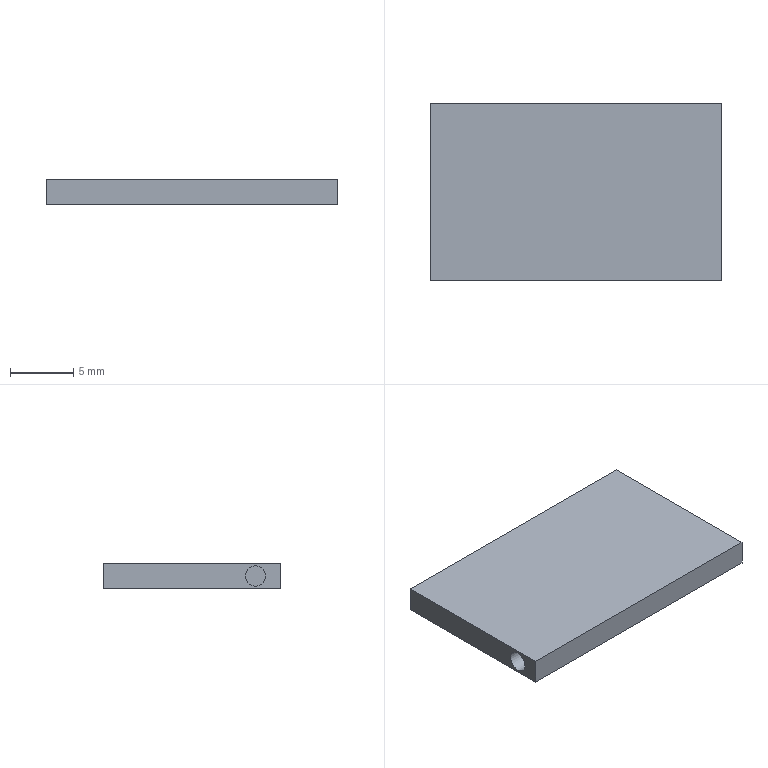Component | NX | CONNECTING_RECT_2 | 1 solid | 10 faces | box 23 x 14 x 2 mm | volume 636 mm3 | plane 8 | cylinder 2 | commonest cylinder face diameters 1.6 x2
STEP:
#1=CARTESIAN_POINT('',(0.,0.,0.));
#2=DIRECTION('',(0.,0.,1.));
#3=DIRECTION('',(1.,0.,0.));
#4=AXIS2_PLACEMENT_3D('',#1,#2,#3);
#5=CARTESIAN_POINT('',(-11.5,-4.375,30.));
#6=VERTEX_POINT('',#5);
#7=CARTESIAN_POINT('',(-11.5,-3.575,30.));
#8=DIRECTION('',(1.,0.,0.));
#9=DIRECTION('',(0.,-1.,0.));
#10=AXIS2_PLACEMENT_3D('',#7,#8,#9);
#11=CIRCLE('',#10,0.8);
#12=CARTESIAN_POINT('',(-11.5,8.425,29.));
#13=DIRECTION('',(-1.,0.,0.));
#14=DIRECTION('',(0.,0.,1.));
#15=AXIS2_PLACEMENT_3D('',#12,#13,#14);
#16=PLANE('',#15);
#17=CARTESIAN_POINT('',(1.,-12.8));
#18=CARTESIAN_POINT('',(-0.3856,-12.8));
#19=CARTESIAN_POINT('',(0.3072,-11.6));
#20=CARTESIAN_POINT('',(1.,-10.4));
#21=CARTESIAN_POINT('',(1.693,-11.6));
#22=CARTESIAN_POINT('',(2.386,-12.8));
#23=CARTESIAN_POINT('',(1.,-12.8));
#24=(BOUNDED_CURVE()B_SPLINE_CURVE(2,(#17,#18,#19,#20,#21,#22,#23),.UNSPECIFIED.,.T.,.F.)B_SPLINE_CURVE_WITH_KNOTS((1,2,2,2,2,1),(-2.094,0.,2.094,4.189,6.283,8.378),.UNSPECIFIED.)CURVE()GEOMETRIC_REPRESENTATION_ITEM()RATIONAL_B_SPLINE_CURVE((1.,0.5,1.,0.5,1.,0.5,1.))REPRESENTATION_ITEM(''));
#25=(GEOMETRIC_REPRESENTATION_CONTEXT(2)PARAMETRIC_REPRESENTATION_CONTEXT()REPRESENTATION_CONTEXT('',''));
#26=DEFINITIONAL_REPRESENTATION('',(#24),#25);
#27=PCURVE('',#16,#26);
#28=CARTESIAN_POINT('',(-9.5,-3.575,30.));
#29=DIRECTION('',(-1.,0.,0.));
#30=DIRECTION('',(0.,0.,1.));
#31=AXIS2_PLACEMENT_3D('',#28,#29,#30);
#32=CYLINDRICAL_SURFACE('',#31,0.8);
#33=CARTESIAN_POINT('',(10.996,2.));
#34=DIRECTION('',(-1.,0.));
#35=VECTOR('',#34,1.);
#36=LINE('',#33,#35);
#37=(GEOMETRIC_REPRESENTATION_CONTEXT(2)PARAMETRIC_REPRESENTATION_CONTEXT()REPRESENTATION_CONTEXT('',''));
#38=DEFINITIONAL_REPRESENTATION('',(#36),#37);
#39=PCURVE('',#32,#38);
#40=SURFACE_CURVE('',#11,(#27,#39),.PCURVE_S1.);
#41=EDGE_CURVE('',#6,#6,#40,.T.);
#42=ORIENTED_EDGE('',*,*,#41,.T.);
#43=EDGE_LOOP('',(#42));
#44=FACE_BOUND('',#43,.T.);
#45=CARTESIAN_POINT('',(-11.5,8.425,31.));
#46=VERTEX_POINT('',#45);
#47=CARTESIAN_POINT('',(-11.5,-5.575,31.));
#48=VERTEX_POINT('',#47);
#49=CARTESIAN_POINT('',(-11.5,8.425,31.));
#50=DIRECTION('',(0.,-1.,0.));
#51=VECTOR('',#50,1.);
#52=LINE('',#49,#51);
#53=CARTESIAN_POINT('',(2.,0.));
#54=DIRECTION('',(0.,-1.));
#55=VECTOR('',#54,1.);
#56=LINE('',#53,#55);
#57=(GEOMETRIC_REPRESENTATION_CONTEXT(2)PARAMETRIC_REPRESENTATION_CONTEXT()REPRESENTATION_CONTEXT('',''));
#58=DEFINITIONAL_REPRESENTATION('',(#56),#57);
#59=PCURVE('',#16,#58);
#60=CARTESIAN_POINT('',(6.5,1.925,31.));
#61=DIRECTION('',(0.,0.,1.));
#62=DIRECTION('',(1.,0.,0.));
#63=AXIS2_PLACEMENT_3D('',#60,#61,#62);
#64=PLANE('',#63);
#65=CARTESIAN_POINT('',(-18.,6.5));
#66=DIRECTION('',(0.,-1.));
#67=VECTOR('',#66,1.);
#68=LINE('',#65,#67);
#69=(GEOMETRIC_REPRESENTATION_CONTEXT(2)PARAMETRIC_REPRESENTATION_CONTEXT()REPRESENTATION_CONTEXT('',''));
#70=DEFINITIONAL_REPRESENTATION('',(#68),#69);
#71=PCURVE('',#64,#70);
#72=SURFACE_CURVE('',#52,(#59,#71),.PCURVE_S1.);
#73=EDGE_CURVE('',#46,#48,#72,.T.);
#74=ORIENTED_EDGE('',*,*,#73,.F.);
#75=CARTESIAN_POINT('',(-11.5,8.425,29.));
#76=VERTEX_POINT('',#75);
#77=CARTESIAN_POINT('',(-11.5,8.425,29.));
#78=DIRECTION('',(0.,0.,1.));
#79=VECTOR('',#78,1.);
#80=LINE('',#77,#79);
#81=CARTESIAN_POINT('',(0.,0.));
#82=DIRECTION('',(1.,0.));
#83=VECTOR('',#82,1.);
#84=LINE('',#81,#83);
#85=(GEOMETRIC_REPRESENTATION_CONTEXT(2)PARAMETRIC_REPRESENTATION_CONTEXT()REPRESENTATION_CONTEXT('',''));
#86=DEFINITIONAL_REPRESENTATION('',(#84),#85);
#87=PCURVE('',#16,#86);
#88=CARTESIAN_POINT('',(11.5,8.425,29.));
#89=DIRECTION('',(-0.,1.,0.));
#90=DIRECTION('',(-1.,-0.,0.));
#91=AXIS2_PLACEMENT_3D('',#88,#89,#90);
#92=PLANE('',#91);
#93=CARTESIAN_POINT('',(23.,0.));
#94=DIRECTION('',(0.,1.));
#95=VECTOR('',#94,1.);
#96=LINE('',#93,#95);
#97=(GEOMETRIC_REPRESENTATION_CONTEXT(2)PARAMETRIC_REPRESENTATION_CONTEXT()REPRESENTATION_CONTEXT('',''));
#98=DEFINITIONAL_REPRESENTATION('',(#96),#97);
#99=PCURVE('',#92,#98);
#100=SURFACE_CURVE('',#80,(#87,#99),.PCURVE_S1.);
#101=EDGE_CURVE('',#76,#46,#100,.T.);
#102=ORIENTED_EDGE('',*,*,#101,.F.);
#103=CARTESIAN_POINT('',(-11.5,-5.575,29.));
#104=VERTEX_POINT('',#103);
#105=CARTESIAN_POINT('',(-11.5,8.425,29.));
#106=DIRECTION('',(0.,-1.,0.));
#107=VECTOR('',#106,1.);
#108=LINE('',#105,#107);
#109=CARTESIAN_POINT('',(0.,0.));
#110=DIRECTION('',(0.,-1.));
#111=VECTOR('',#110,1.);
#112=LINE('',#109,#111);
#113=(GEOMETRIC_REPRESENTATION_CONTEXT(2)PARAMETRIC_REPRESENTATION_CONTEXT()REPRESENTATION_CONTEXT('',''));
#114=DEFINITIONAL_REPRESENTATION('',(#112),#113);
#115=PCURVE('',#16,#114);
#116=CARTESIAN_POINT('',(6.5,1.925,29.));
#117=DIRECTION('',(0.,0.,1.));
#118=DIRECTION('',(1.,0.,0.));
#119=AXIS2_PLACEMENT_3D('',#116,#117,#118);
#120=PLANE('',#119);
#121=CARTESIAN_POINT('',(-18.,6.5));
#122=DIRECTION('',(0.,-1.));
#123=VECTOR('',#122,1.);
#124=LINE('',#121,#123);
#125=(GEOMETRIC_REPRESENTATION_CONTEXT(2)PARAMETRIC_REPRESENTATION_CONTEXT()REPRESENTATION_CONTEXT('',''));
#126=DEFINITIONAL_REPRESENTATION('',(#124),#125);
#127=PCURVE('',#120,#126);
#128=SURFACE_CURVE('',#108,(#115,#127),.PCURVE_S1.);
#129=EDGE_CURVE('',#76,#104,#128,.T.);
#130=ORIENTED_EDGE('',*,*,#129,.T.);
#131=CARTESIAN_POINT('',(-11.5,-5.575,29.));
#132=DIRECTION('',(0.,0.,1.));
#133=VECTOR('',#132,1.);
#134=LINE('',#131,#133);
#135=CARTESIAN_POINT('',(0.,-14.));
#136=DIRECTION('',(1.,0.));
#137=VECTOR('',#136,1.);
#138=LINE('',#135,#137);
#139=(GEOMETRIC_REPRESENTATION_CONTEXT(2)PARAMETRIC_REPRESENTATION_CONTEXT()REPRESENTATION_CONTEXT('',''));
#140=DEFINITIONAL_REPRESENTATION('',(#138),#139);
#141=PCURVE('',#16,#140);
#142=CARTESIAN_POINT('',(-11.5,-5.575,29.));
#143=DIRECTION('',(0.,-1.,0.));
#144=DIRECTION('',(1.,0.,0.));
#145=AXIS2_PLACEMENT_3D('',#142,#143,#144);
#146=PLANE('',#145);
#147=CARTESIAN_POINT('',(0.,0.));
#148=DIRECTION('',(0.,1.));
#149=VECTOR('',#148,1.);
#150=LINE('',#147,#149);
#151=(GEOMETRIC_REPRESENTATION_CONTEXT(2)PARAMETRIC_REPRESENTATION_CONTEXT()REPRESENTATION_CONTEXT('',''));
#152=DEFINITIONAL_REPRESENTATION('',(#150),#151);
#153=PCURVE('',#146,#152);
#154=SURFACE_CURVE('',#134,(#141,#153),.PCURVE_S1.);
#155=EDGE_CURVE('',#104,#48,#154,.T.);
#156=ORIENTED_EDGE('',*,*,#155,.T.);
#157=EDGE_LOOP('',(#74,#102,#130,#156));
#158=FACE_BOUND('',#157,.T.);
#159=ADVANCED_FACE('',(#44,#158),#16,.T.);
#160=CARTESIAN_POINT('',(11.5,-5.575,31.));
#161=VERTEX_POINT('',#160);
#162=CARTESIAN_POINT('',(-11.5,-5.575,31.));
#163=DIRECTION('',(1.,0.,0.));
#164=VECTOR('',#163,1.);
#165=LINE('',#162,#164);
#166=CARTESIAN_POINT('',(0.,2.));
#167=DIRECTION('',(1.,0.));
#168=VECTOR('',#167,1.);
#169=LINE('',#166,#168);
#170=(GEOMETRIC_REPRESENTATION_CONTEXT(2)PARAMETRIC_REPRESENTATION_CONTEXT()REPRESENTATION_CONTEXT('',''));
#171=DEFINITIONAL_REPRESENTATION('',(#169),#170);
#172=PCURVE('',#146,#171);
#173=CARTESIAN_POINT('',(-18.,-7.5));
#174=DIRECTION('',(1.,0.));
#175=VECTOR('',#174,1.);
#176=LINE('',#173,#175);
#177=(GEOMETRIC_REPRESENTATION_CONTEXT(2)PARAMETRIC_REPRESENTATION_CONTEXT()REPRESENTATION_CONTEXT('',''));
#178=DEFINITIONAL_REPRESENTATION('',(#176),#177);
#179=PCURVE('',#64,#178);
#180=SURFACE_CURVE('',#165,(#172,#179),.PCURVE_S1.);
#181=EDGE_CURVE('',#48,#161,#180,.T.);
#182=ORIENTED_EDGE('',*,*,#181,.F.);
#183=ORIENTED_EDGE('',*,*,#155,.F.);
#184=CARTESIAN_POINT('',(11.5,-5.575,29.));
#185=VERTEX_POINT('',#184);
#186=CARTESIAN_POINT('',(-11.5,-5.575,29.));
#187=DIRECTION('',(1.,0.,0.));
#188=VECTOR('',#187,1.);
#189=LINE('',#186,#188);
#190=CARTESIAN_POINT('',(0.,0.));
#191=DIRECTION('',(1.,0.));
#192=VECTOR('',#191,1.);
#193=LINE('',#190,#192);
#194=(GEOMETRIC_REPRESENTATION_CONTEXT(2)PARAMETRIC_REPRESENTATION_CONTEXT()REPRESENTATION_CONTEXT('',''));
#195=DEFINITIONAL_REPRESENTATION('',(#193),#194);
#196=PCURVE('',#146,#195);
#197=CARTESIAN_POINT('',(-18.,-7.5));
#198=DIRECTION('',(1.,0.));
#199=VECTOR('',#198,1.);
#200=LINE('',#197,#199);
#201=(GEOMETRIC_REPRESENTATION_CONTEXT(2)PARAMETRIC_REPRESENTATION_CONTEXT()REPRESENTATION_CONTEXT('',''));
#202=DEFINITIONAL_REPRESENTATION('',(#200),#201);
#203=PCURVE('',#120,#202);
#204=SURFACE_CURVE('',#189,(#196,#203),.PCURVE_S1.);
#205=EDGE_CURVE('',#104,#185,#204,.T.);
#206=ORIENTED_EDGE('',*,*,#205,.T.);
#207=CARTESIAN_POINT('',(11.5,-5.575,29.));
#208=DIRECTION('',(0.,0.,1.));
#209=VECTOR('',#208,1.);
#210=LINE('',#207,#209);
#211=CARTESIAN_POINT('',(23.,0.));
#212=DIRECTION('',(0.,1.));
#213=VECTOR('',#212,1.);
#214=LINE('',#211,#213);
#215=(GEOMETRIC_REPRESENTATION_CONTEXT(2)PARAMETRIC_REPRESENTATION_CONTEXT()REPRESENTATION_CONTEXT('',''));
#216=DEFINITIONAL_REPRESENTATION('',(#214),#215);
#217=PCURVE('',#146,#216);
#218=CARTESIAN_POINT('',(11.5,-5.575,29.));
#219=DIRECTION('',(1.,0.,0.));
#220=DIRECTION('',(-0.,1.,0.));
#221=AXIS2_PLACEMENT_3D('',#218,#219,#220);
#222=PLANE('',#221);
#223=CARTESIAN_POINT('',(0.,0.));
#224=DIRECTION('',(0.,1.));
#225=VECTOR('',#224,1.);
#226=LINE('',#223,#225);
#227=(GEOMETRIC_REPRESENTATION_CONTEXT(2)PARAMETRIC_REPRESENTATION_CONTEXT()REPRESENTATION_CONTEXT('',''));
#228=DEFINITIONAL_REPRESENTATION('',(#226),#227);
#229=PCURVE('',#222,#228);
#230=SURFACE_CURVE('',#210,(#217,#229),.PCURVE_S1.);
#231=EDGE_CURVE('',#185,#161,#230,.T.);
#232=ORIENTED_EDGE('',*,*,#231,.T.);
#233=EDGE_LOOP('',(#182,#183,#206,#232));
#234=FACE_BOUND('',#233,.T.);
#235=ADVANCED_FACE('',(#234),#146,.T.);
#236=CARTESIAN_POINT('',(11.5,7.225,30.));
#237=VERTEX_POINT('',#236);
#238=CARTESIAN_POINT('',(11.5,6.425,30.));
#239=DIRECTION('',(1.,0.,0.));
#240=DIRECTION('',(0.,1.,0.));
#241=AXIS2_PLACEMENT_3D('',#238,#239,#240);
#242=CIRCLE('',#241,0.8);
#243=CARTESIAN_POINT('',(12.,1.));
#244=DIRECTION('',(1.,0.));
#245=AXIS2_PLACEMENT_2D('',#243,#244);
#246=CIRCLE('',#245,0.8);
#247=(GEOMETRIC_REPRESENTATION_CONTEXT(2)PARAMETRIC_REPRESENTATION_CONTEXT()REPRESENTATION_CONTEXT('',''));
#248=DEFINITIONAL_REPRESENTATION('',(#246),#247);
#249=PCURVE('',#222,#248);
#250=CARTESIAN_POINT('',(9.5,6.425,30.));
#251=DIRECTION('',(1.,0.,0.));
#252=DIRECTION('',(0.,0.,-1.));
#253=AXIS2_PLACEMENT_3D('',#250,#251,#252);
#254=CYLINDRICAL_SURFACE('',#253,0.8);
#255=CARTESIAN_POINT('',(1.571,2.));
#256=DIRECTION('',(1.,0.));
#257=VECTOR('',#256,1.);
#258=LINE('',#255,#257);
#259=(GEOMETRIC_REPRESENTATION_CONTEXT(2)PARAMETRIC_REPRESENTATION_CONTEXT()REPRESENTATION_CONTEXT('',''));
#260=DEFINITIONAL_REPRESENTATION('',(#258),#259);
#261=PCURVE('',#254,#260);
#262=SURFACE_CURVE('',#242,(#249,#261),.PCURVE_S1.);
#263=EDGE_CURVE('',#237,#237,#262,.T.);
#264=ORIENTED_EDGE('',*,*,#263,.F.);
#265=EDGE_LOOP('',(#264));
#266=FACE_BOUND('',#265,.T.);
#267=CARTESIAN_POINT('',(11.5,8.425,31.));
#268=VERTEX_POINT('',#267);
#269=CARTESIAN_POINT('',(11.5,-5.575,31.));
#270=DIRECTION('',(-0.,1.,0.));
#271=VECTOR('',#270,1.);
#272=LINE('',#269,#271);
#273=CARTESIAN_POINT('',(0.,2.));
#274=DIRECTION('',(1.,0.));
#275=VECTOR('',#274,1.);
#276=LINE('',#273,#275);
#277=(GEOMETRIC_REPRESENTATION_CONTEXT(2)PARAMETRIC_REPRESENTATION_CONTEXT()REPRESENTATION_CONTEXT('',''));
#278=DEFINITIONAL_REPRESENTATION('',(#276),#277);
#279=PCURVE('',#222,#278);
#280=CARTESIAN_POINT('',(5.,-7.5));
#281=DIRECTION('',(-0.,1.));
#282=VECTOR('',#281,1.);
#283=LINE('',#280,#282);
#284=(GEOMETRIC_REPRESENTATION_CONTEXT(2)PARAMETRIC_REPRESENTATION_CONTEXT()REPRESENTATION_CONTEXT('',''));
#285=DEFINITIONAL_REPRESENTATION('',(#283),#284);
#286=PCURVE('',#64,#285);
#287=SURFACE_CURVE('',#272,(#279,#286),.PCURVE_S1.);
#288=EDGE_CURVE('',#161,#268,#287,.T.);
#289=ORIENTED_EDGE('',*,*,#288,.F.);
#290=ORIENTED_EDGE('',*,*,#231,.F.);
#291=CARTESIAN_POINT('',(11.5,8.425,29.));
#292=VERTEX_POINT('',#291);
#293=CARTESIAN_POINT('',(11.5,-5.575,29.));
#294=DIRECTION('',(-0.,1.,0.));
#295=VECTOR('',#294,1.);
#296=LINE('',#293,#295);
#297=CARTESIAN_POINT('',(0.,0.));
#298=DIRECTION('',(1.,0.));
#299=VECTOR('',#298,1.);
#300=LINE('',#297,#299);
#301=(GEOMETRIC_REPRESENTATION_CONTEXT(2)PARAMETRIC_REPRESENTATION_CONTEXT()REPRESENTATION_CONTEXT('',''));
#302=DEFINITIONAL_REPRESENTATION('',(#300),#301);
#303=PCURVE('',#222,#302);
#304=CARTESIAN_POINT('',(5.,-7.5));
#305=DIRECTION('',(-0.,1.));
#306=VECTOR('',#305,1.);
#307=LINE('',#304,#306);
#308=(GEOMETRIC_REPRESENTATION_CONTEXT(2)PARAMETRIC_REPRESENTATION_CONTEXT()REPRESENTATION_CONTEXT('',''));
#309=DEFINITIONAL_REPRESENTATION('',(#307),#308);
#310=PCURVE('',#120,#309);
#311=SURFACE_CURVE('',#296,(#303,#310),.PCURVE_S1.);
#312=EDGE_CURVE('',#185,#292,#311,.T.);
#313=ORIENTED_EDGE('',*,*,#312,.T.);
#314=CARTESIAN_POINT('',(11.5,8.425,29.));
#315=DIRECTION('',(0.,0.,1.));
#316=VECTOR('',#315,1.);
#317=LINE('',#314,#316);
#318=CARTESIAN_POINT('',(14.,0.));
#319=DIRECTION('',(0.,1.));
#320=VECTOR('',#319,1.);
#321=LINE('',#318,#320);
#322=(GEOMETRIC_REPRESENTATION_CONTEXT(2)PARAMETRIC_REPRESENTATION_CONTEXT()REPRESENTATION_CONTEXT('',''));
#323=DEFINITIONAL_REPRESENTATION('',(#321),#322);
#324=PCURVE('',#222,#323);
#325=CARTESIAN_POINT('',(0.,0.));
#326=DIRECTION('',(0.,1.));
#327=VECTOR('',#326,1.);
#328=LINE('',#325,#327);
#329=(GEOMETRIC_REPRESENTATION_CONTEXT(2)PARAMETRIC_REPRESENTATION_CONTEXT()REPRESENTATION_CONTEXT('',''));
#330=DEFINITIONAL_REPRESENTATION('',(#328),#329);
#331=PCURVE('',#92,#330);
#332=SURFACE_CURVE('',#317,(#324,#331),.PCURVE_S1.);
#333=EDGE_CURVE('',#292,#268,#332,.T.);
#334=ORIENTED_EDGE('',*,*,#333,.T.);
#335=EDGE_LOOP('',(#289,#290,#313,#334));
#336=FACE_BOUND('',#335,.T.);
#337=ADVANCED_FACE('',(#266,#336),#222,.T.);
#338=CARTESIAN_POINT('',(11.5,8.425,31.));
#339=DIRECTION('',(-1.,-0.,0.));
#340=VECTOR('',#339,1.);
#341=LINE('',#338,#340);
#342=CARTESIAN_POINT('',(0.,2.));
#343=DIRECTION('',(1.,0.));
#344=VECTOR('',#343,1.);
#345=LINE('',#342,#344);
#346=(GEOMETRIC_REPRESENTATION_CONTEXT(2)PARAMETRIC_REPRESENTATION_CONTEXT()REPRESENTATION_CONTEXT('',''));
#347=DEFINITIONAL_REPRESENTATION('',(#345),#346);
#348=PCURVE('',#92,#347);
#349=CARTESIAN_POINT('',(5.,6.5));
#350=DIRECTION('',(-1.,-0.));
#351=VECTOR('',#350,1.);
#352=LINE('',#349,#351);
#353=(GEOMETRIC_REPRESENTATION_CONTEXT(2)PARAMETRIC_REPRESENTATION_CONTEXT()REPRESENTATION_CONTEXT('',''));
#354=DEFINITIONAL_REPRESENTATION('',(#352),#353);
#355=PCURVE('',#64,#354);
#356=SURFACE_CURVE('',#341,(#348,#355),.PCURVE_S1.);
#357=EDGE_CURVE('',#268,#46,#356,.T.);
#358=ORIENTED_EDGE('',*,*,#357,.F.);
#359=ORIENTED_EDGE('',*,*,#333,.F.);
#360=CARTESIAN_POINT('',(11.5,8.425,29.));
#361=DIRECTION('',(-1.,-0.,0.));
#362=VECTOR('',#361,1.);
#363=LINE('',#360,#362);
#364=CARTESIAN_POINT('',(0.,0.));
#365=DIRECTION('',(1.,0.));
#366=VECTOR('',#365,1.);
#367=LINE('',#364,#366);
#368=(GEOMETRIC_REPRESENTATION_CONTEXT(2)PARAMETRIC_REPRESENTATION_CONTEXT()REPRESENTATION_CONTEXT('',''));
#369=DEFINITIONAL_REPRESENTATION('',(#367),#368);
#370=PCURVE('',#92,#369);
#371=CARTESIAN_POINT('',(5.,6.5));
#372=DIRECTION('',(-1.,-0.));
#373=VECTOR('',#372,1.);
#374=LINE('',#371,#373);
#375=(GEOMETRIC_REPRESENTATION_CONTEXT(2)PARAMETRIC_REPRESENTATION_CONTEXT()REPRESENTATION_CONTEXT('',''));
#376=DEFINITIONAL_REPRESENTATION('',(#374),#375);
#377=PCURVE('',#120,#376);
#378=SURFACE_CURVE('',#363,(#370,#377),.PCURVE_S1.);
#379=EDGE_CURVE('',#292,#76,#378,.T.);
#380=ORIENTED_EDGE('',*,*,#379,.T.);
#381=ORIENTED_EDGE('',*,*,#101,.T.);
#382=EDGE_LOOP('',(#358,#359,#380,#381));
#383=FACE_BOUND('',#382,.T.);
#384=ADVANCED_FACE('',(#383),#92,.T.);
#385=ORIENTED_EDGE('',*,*,#129,.F.);
#386=ORIENTED_EDGE('',*,*,#379,.F.);
#387=ORIENTED_EDGE('',*,*,#312,.F.);
#388=ORIENTED_EDGE('',*,*,#205,.F.);
#389=EDGE_LOOP('',(#385,#386,#387,#388));
#390=FACE_BOUND('',#389,.T.);
#391=ADVANCED_FACE('',(#390),#120,.F.);
#392=ORIENTED_EDGE('',*,*,#73,.T.);
#393=ORIENTED_EDGE('',*,*,#181,.T.);
#394=ORIENTED_EDGE('',*,*,#288,.T.);
#395=ORIENTED_EDGE('',*,*,#357,.T.);
#396=EDGE_LOOP('',(#392,#393,#394,#395));
#397=FACE_BOUND('',#396,.T.);
#398=ADVANCED_FACE('',(#397),#64,.T.);
#399=CARTESIAN_POINT('',(9.5,7.225,30.));
#400=VERTEX_POINT('',#399);
#401=CARTESIAN_POINT('',(9.5,6.425,30.));
#402=DIRECTION('',(1.,0.,0.));
#403=DIRECTION('',(0.,1.,0.));
#404=AXIS2_PLACEMENT_3D('',#401,#402,#403);
#405=CIRCLE('',#404,0.8);
#406=CARTESIAN_POINT('',(1.571,0.));
#407=DIRECTION('',(1.,0.));
#408=VECTOR('',#407,1.);
#409=LINE('',#406,#408);
#410=(GEOMETRIC_REPRESENTATION_CONTEXT(2)PARAMETRIC_REPRESENTATION_CONTEXT()REPRESENTATION_CONTEXT('',''));
#411=DEFINITIONAL_REPRESENTATION('',(#409),#410);
#412=PCURVE('',#254,#411);
#413=CARTESIAN_POINT('',(9.5,6.425,30.));
#414=DIRECTION('',(-1.,0.,0.));
#415=DIRECTION('',(0.,0.,1.));
#416=AXIS2_PLACEMENT_3D('',#413,#414,#415);
#417=PLANE('',#416);
#418=CARTESIAN_POINT('',(0.,0.8));
#419=CARTESIAN_POINT('',(1.386,0.8));
#420=CARTESIAN_POINT('',(0.6928,-0.4));
#421=CARTESIAN_POINT('',(0.,-1.6));
#422=CARTESIAN_POINT('',(-0.6928,-0.4));
#423=CARTESIAN_POINT('',(-1.386,0.8));
#424=CARTESIAN_POINT('',(0.,0.8));
#425=(BOUNDED_CURVE()B_SPLINE_CURVE(2,(#418,#419,#420,#421,#422,#423,#424),.UNSPECIFIED.,.T.,.F.)B_SPLINE_CURVE_WITH_KNOTS((1,2,2,2,2,1),(-2.094,0.,2.094,4.189,6.283,8.378),.UNSPECIFIED.)CURVE()GEOMETRIC_REPRESENTATION_ITEM()RATIONAL_B_SPLINE_CURVE((1.,0.5,1.,0.5,1.,0.5,1.))REPRESENTATION_ITEM(''));
#426=(GEOMETRIC_REPRESENTATION_CONTEXT(2)PARAMETRIC_REPRESENTATION_CONTEXT()REPRESENTATION_CONTEXT('',''));
#427=DEFINITIONAL_REPRESENTATION('',(#425),#426);
#428=PCURVE('',#417,#427);
#429=SURFACE_CURVE('',#405,(#412,#428),.PCURVE_S1.);
#430=EDGE_CURVE('',#400,#400,#429,.T.);
#431=ORIENTED_EDGE('',*,*,#430,.T.);
#432=CARTESIAN_POINT('',(9.5,7.225,30.));
#433=CARTESIAN_POINT('',(11.5,7.225,30.));
#434=B_SPLINE_CURVE_WITH_KNOTS('',1,(#432,#433),.UNSPECIFIED.,.F.,.F.,(2,2),(0.,2.),.PIECEWISE_BEZIER_KNOTS.);
#435=CARTESIAN_POINT('',(7.854,0.));
#436=DIRECTION('',(0.,1.));
#437=VECTOR('',#436,1.);
#438=LINE('',#435,#437);
#439=(GEOMETRIC_REPRESENTATION_CONTEXT(2)PARAMETRIC_REPRESENTATION_CONTEXT()REPRESENTATION_CONTEXT('',''));
#440=DEFINITIONAL_REPRESENTATION('',(#438),#439);
#441=PCURVE('',#254,#440);
#442=CARTESIAN_POINT('',(1.571,0.));
#443=DIRECTION('',(0.,1.));
#444=VECTOR('',#443,1.);
#445=LINE('',#442,#444);
#446=(GEOMETRIC_REPRESENTATION_CONTEXT(2)PARAMETRIC_REPRESENTATION_CONTEXT()REPRESENTATION_CONTEXT('',''));
#447=DEFINITIONAL_REPRESENTATION('',(#445),#446);
#448=PCURVE('',#254,#447);
#449=SEAM_CURVE('',#434,(#441,#448),.PCURVE_S1.);
#450=EDGE_CURVE('',#400,#237,#449,.T.);
#451=ORIENTED_EDGE('',*,*,#450,.T.);
#452=ORIENTED_EDGE('',*,*,#263,.F.);
#453=ORIENTED_EDGE('',*,*,#450,.F.);
#454=EDGE_LOOP('',(#431,#451,#452,#453));
#455=FACE_BOUND('',#454,.F.);
#456=ADVANCED_FACE('',(#455),#254,.F.);
#457=ORIENTED_EDGE('',*,*,#430,.T.);
#458=EDGE_LOOP('',(#457));
#459=FACE_BOUND('',#458,.T.);
#460=ADVANCED_FACE('',(#459),#417,.F.);
#461=CARTESIAN_POINT('',(-9.5,-4.375,30.));
#462=VERTEX_POINT('',#461);
#463=CARTESIAN_POINT('',(-9.5,-3.575,30.));
#464=DIRECTION('',(-1.,0.,0.));
#465=DIRECTION('',(0.,-1.,0.));
#466=AXIS2_PLACEMENT_3D('',#463,#464,#465);
#467=CIRCLE('',#466,0.8);
#468=CARTESIAN_POINT('',(4.712,0.));
#469=DIRECTION('',(1.,0.));
#470=VECTOR('',#469,1.);
#471=LINE('',#468,#470);
#472=(GEOMETRIC_REPRESENTATION_CONTEXT(2)PARAMETRIC_REPRESENTATION_CONTEXT()REPRESENTATION_CONTEXT('',''));
#473=DEFINITIONAL_REPRESENTATION('',(#471),#472);
#474=PCURVE('',#32,#473);
#475=CARTESIAN_POINT('',(-9.5,-3.575,30.));
#476=DIRECTION('',(1.,0.,0.));
#477=DIRECTION('',(0.,0.,-1.));
#478=AXIS2_PLACEMENT_3D('',#475,#476,#477);
#479=PLANE('',#478);
#480=CARTESIAN_POINT('',(0.,-0.8));
#481=CARTESIAN_POINT('',(-1.386,-0.8));
#482=CARTESIAN_POINT('',(-0.6928,0.4));
#483=CARTESIAN_POINT('',(-0.,1.6));
#484=CARTESIAN_POINT('',(0.6928,0.4));
#485=CARTESIAN_POINT('',(1.386,-0.8));
#486=CARTESIAN_POINT('',(0.,-0.8));
#487=(BOUNDED_CURVE()B_SPLINE_CURVE(2,(#480,#481,#482,#483,#484,#485,#486),.UNSPECIFIED.,.T.,.F.)B_SPLINE_CURVE_WITH_KNOTS((1,2,2,2,2,1),(-2.094,0.,2.094,4.189,6.283,8.378),.UNSPECIFIED.)CURVE()GEOMETRIC_REPRESENTATION_ITEM()RATIONAL_B_SPLINE_CURVE((1.,0.5,1.,0.5,1.,0.5,1.))REPRESENTATION_ITEM(''));
#488=(GEOMETRIC_REPRESENTATION_CONTEXT(2)PARAMETRIC_REPRESENTATION_CONTEXT()REPRESENTATION_CONTEXT('',''));
#489=DEFINITIONAL_REPRESENTATION('',(#487),#488);
#490=PCURVE('',#479,#489);
#491=SURFACE_CURVE('',#467,(#474,#490),.PCURVE_S1.);
#492=EDGE_CURVE('',#462,#462,#491,.T.);
#493=ORIENTED_EDGE('',*,*,#492,.T.);
#494=CARTESIAN_POINT('',(-9.5,-4.375,30.));
#495=CARTESIAN_POINT('',(-11.5,-4.375,30.));
#496=B_SPLINE_CURVE_WITH_KNOTS('',1,(#494,#495),.UNSPECIFIED.,.F.,.F.,(2,2),(0.,2.),.PIECEWISE_BEZIER_KNOTS.);
#497=CARTESIAN_POINT('',(10.996,0.));
#498=DIRECTION('',(0.,1.));
#499=VECTOR('',#498,1.);
#500=LINE('',#497,#499);
#501=(GEOMETRIC_REPRESENTATION_CONTEXT(2)PARAMETRIC_REPRESENTATION_CONTEXT()REPRESENTATION_CONTEXT('',''));
#502=DEFINITIONAL_REPRESENTATION('',(#500),#501);
#503=PCURVE('',#32,#502);
#504=CARTESIAN_POINT('',(4.712,0.));
#505=DIRECTION('',(0.,1.));
#506=VECTOR('',#505,1.);
#507=LINE('',#504,#506);
#508=(GEOMETRIC_REPRESENTATION_CONTEXT(2)PARAMETRIC_REPRESENTATION_CONTEXT()REPRESENTATION_CONTEXT('',''));
#509=DEFINITIONAL_REPRESENTATION('',(#507),#508);
#510=PCURVE('',#32,#509);
#511=SEAM_CURVE('',#496,(#503,#510),.PCURVE_S1.);
#512=EDGE_CURVE('',#462,#6,#511,.T.);
#513=ORIENTED_EDGE('',*,*,#512,.T.);
#514=ORIENTED_EDGE('',*,*,#41,.T.);
#515=ORIENTED_EDGE('',*,*,#512,.F.);
#516=EDGE_LOOP('',(#493,#513,#514,#515));
#517=FACE_BOUND('',#516,.F.);
#518=ADVANCED_FACE('',(#517),#32,.F.);
#519=ORIENTED_EDGE('',*,*,#492,.T.);
#520=EDGE_LOOP('',(#519));
#521=FACE_BOUND('',#520,.T.);
#522=ADVANCED_FACE('',(#521),#479,.F.);
#523=CLOSED_SHELL('',(#159,#235,#337,#384,#391,#398,#456,#460,#518,#522));
#524=MANIFOLD_SOLID_BREP('',#523);
#525=(LENGTH_UNIT()NAMED_UNIT(*)SI_UNIT(.MILLI.,.METRE.));
#526=UNCERTAINTY_MEASURE_WITH_UNIT(LENGTH_MEASURE(0.000002),#525,'','');
#527=(NAMED_UNIT(*)PLANE_ANGLE_UNIT()SI_UNIT($,.RADIAN.));
#528=(NAMED_UNIT(*)SI_UNIT($,.STERADIAN.)SOLID_ANGLE_UNIT());
#529=(GEOMETRIC_REPRESENTATION_CONTEXT(3)GLOBAL_UNCERTAINTY_ASSIGNED_CONTEXT((#526))GLOBAL_UNIT_ASSIGNED_CONTEXT((#525,#527,#528))REPRESENTATION_CONTEXT('',''));
#530=ADVANCED_BREP_SHAPE_REPRESENTATION('',(#4,#524),#529);